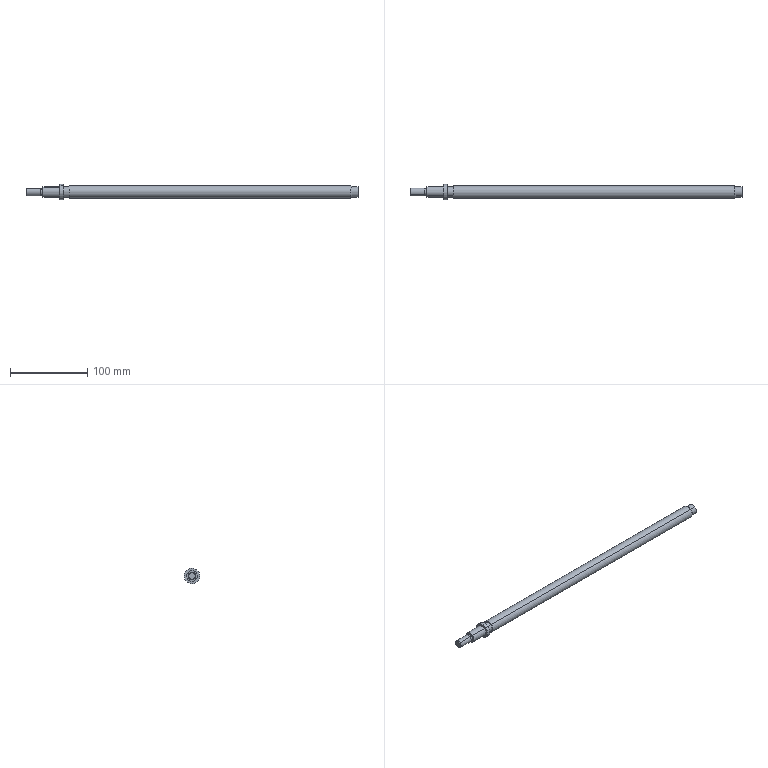Component | SolidWorks | 32FineAdjustmentLeadScrew-1 | 1 solid | 26 faces | box 430 x 20 x 20 mm | volume 81961 mm3 | cylinder 14 | plane 8 | cone 4 | commonest cylinder face diameters 13 x4 10 x2 8 x2 14 x2 20 x2 16 x2
STEP:
#1=COLOUR_RGB('',0.7922,0.8196,0.9333);
#2=FILL_AREA_STYLE_COLOUR('',#1);
#3=FILL_AREA_STYLE('',(#2));
#4=SURFACE_STYLE_FILL_AREA(#3);
#5=SURFACE_SIDE_STYLE('',(#4));
#6=SURFACE_STYLE_USAGE(.BOTH.,#5);
#7=PRESENTATION_STYLE_ASSIGNMENT((#6));
#8=CARTESIAN_POINT('',(7.008,2.405,-4.648));
#9=VERTEX_POINT('',#8);
#10=CARTESIAN_POINT('',(7.008,2.083,-4.25));
#11=VERTEX_POINT('',#10);
#12=CARTESIAN_POINT('',(7.008,2.244,-4.449));
#13=DIRECTION('',(-1.,-0.,0.));
#14=DIRECTION('',(0.,0.6286,-0.7777));
#15=AXIS2_PLACEMENT_3D('',#12,#13,#14);
#16=CIRCLE('',#15,0.2559);
#17=EDGE_CURVE('',#9,#11,#16,.T.);
#18=ORIENTED_EDGE('',*,*,#17,.F.);
#19=CARTESIAN_POINT('',(7.323,2.405,-4.648));
#20=VERTEX_POINT('',#19);
#21=CARTESIAN_POINT('',(7.008,2.405,-4.648));
#22=DIRECTION('',(1.,0.,-0.));
#23=VECTOR('',#22,39.37);
#24=LINE('',#21,#23);
#25=EDGE_CURVE('',#9,#20,#24,.T.);
#26=ORIENTED_EDGE('',*,*,#25,.T.);
#27=CARTESIAN_POINT('',(7.323,2.083,-4.25));
#28=VERTEX_POINT('',#27);
#29=CARTESIAN_POINT('',(7.323,2.244,-4.449));
#30=DIRECTION('',(-1.,-0.,0.));
#31=DIRECTION('',(0.,0.6286,-0.7777));
#32=AXIS2_PLACEMENT_3D('',#29,#30,#31);
#33=CIRCLE('',#32,0.2559);
#34=EDGE_CURVE('',#20,#28,#33,.T.);
#35=ORIENTED_EDGE('',*,*,#34,.T.);
#36=CARTESIAN_POINT('',(7.008,2.083,-4.25));
#37=DIRECTION('',(1.,0.,-0.));
#38=VECTOR('',#37,39.37);
#39=LINE('',#36,#38);
#40=EDGE_CURVE('',#11,#28,#39,.T.);
#41=ORIENTED_EDGE('',*,*,#40,.F.);
#42=EDGE_LOOP('',(#18,#26,#35,#41));
#43=FACE_OUTER_BOUND('',#42,.T.);
#44=CARTESIAN_POINT('',(7.008,2.244,-4.449));
#45=DIRECTION('',(1.,0.,-0.));
#46=DIRECTION('',(0.,-0.6286,0.7777));
#47=AXIS2_PLACEMENT_3D('',#44,#45,#46);
#48=CYLINDRICAL_SURFACE('',#47,0.2559);
#49=ADVANCED_FACE('',(#43),#48,.T.);
#50=CARTESIAN_POINT('',(7.008,2.415,-4.661));
#51=VERTEX_POINT('',#50);
#52=CARTESIAN_POINT('',(7.008,2.073,-4.237));
#53=VERTEX_POINT('',#52);
#54=CARTESIAN_POINT('',(7.008,2.244,-4.449));
#55=DIRECTION('',(-1.,-0.,0.));
#56=DIRECTION('',(0.,0.6286,-0.7777));
#57=AXIS2_PLACEMENT_3D('',#54,#55,#56);
#58=CIRCLE('',#57,0.2723);
#59=EDGE_CURVE('',#51,#53,#58,.T.);
#60=ORIENTED_EDGE('',*,*,#59,.T.);
#61=CARTESIAN_POINT('',(6.965,2.046,-4.204));
#62=VERTEX_POINT('',#61);
#63=CARTESIAN_POINT('',(7.008,2.073,-4.237));
#64=DIRECTION('',(-0.7071,-0.4445,0.5499));
#65=VECTOR('',#64,39.37);
#66=LINE('',#63,#65);
#67=EDGE_CURVE('',#53,#62,#66,.T.);
#68=ORIENTED_EDGE('',*,*,#67,.T.);
#69=CARTESIAN_POINT('',(6.965,2.442,-4.694));
#70=VERTEX_POINT('',#69);
#71=CARTESIAN_POINT('',(6.965,2.244,-4.449));
#72=DIRECTION('',(-1.,-0.,0.));
#73=DIRECTION('',(0.,0.6286,-0.7777));
#74=AXIS2_PLACEMENT_3D('',#71,#72,#73);
#75=CIRCLE('',#74,0.315);
#76=EDGE_CURVE('',#70,#62,#75,.T.);
#77=ORIENTED_EDGE('',*,*,#76,.F.);
#78=CARTESIAN_POINT('',(7.008,2.415,-4.661));
#79=DIRECTION('',(-0.7071,0.4445,-0.5499));
#80=VECTOR('',#79,39.37);
#81=LINE('',#78,#80);
#82=EDGE_CURVE('',#51,#70,#81,.T.);
#83=ORIENTED_EDGE('',*,*,#82,.F.);
#84=EDGE_LOOP('',(#60,#68,#77,#83));
#85=FACE_OUTER_BOUND('',#84,.T.);
#86=CARTESIAN_POINT('',(7.008,2.244,-4.449));
#87=DIRECTION('',(-1.,-0.,0.));
#88=DIRECTION('',(0.,0.6286,-0.7777));
#89=AXIS2_PLACEMENT_3D('',#86,#87,#88);
#90=CONICAL_SURFACE('',#89,0.2723,0.7854);
#91=ADVANCED_FACE('',(#85),#90,.T.);
#92=CARTESIAN_POINT('',(-9.606,2.14,-4.321));
#93=VERTEX_POINT('',#92);
#94=CARTESIAN_POINT('',(-9.606,2.348,-4.577));
#95=VERTEX_POINT('',#94);
#96=CARTESIAN_POINT('',(-9.606,2.244,-4.449));
#97=DIRECTION('',(1.,0.,-0.));
#98=DIRECTION('',(0.,-0.6286,0.7777));
#99=AXIS2_PLACEMENT_3D('',#96,#97,#98);
#100=CIRCLE('',#99,0.1649);
#101=EDGE_CURVE('',#93,#95,#100,.T.);
#102=ORIENTED_EDGE('',*,*,#101,.T.);
#103=CARTESIAN_POINT('',(-9.574,2.368,-4.602));
#104=VERTEX_POINT('',#103);
#105=CARTESIAN_POINT('',(-9.606,2.348,-4.577));
#106=DIRECTION('',(0.7071,0.4445,-0.5499));
#107=VECTOR('',#106,39.37);
#108=LINE('',#105,#107);
#109=EDGE_CURVE('',#95,#104,#108,.T.);
#110=ORIENTED_EDGE('',*,*,#109,.T.);
#111=CARTESIAN_POINT('',(-9.574,2.12,-4.296));
#112=VERTEX_POINT('',#111);
#113=CARTESIAN_POINT('',(-9.574,2.244,-4.449));
#114=DIRECTION('',(1.,0.,-0.));
#115=DIRECTION('',(0.,-0.6286,0.7777));
#116=AXIS2_PLACEMENT_3D('',#113,#114,#115);
#117=CIRCLE('',#116,0.1969);
#118=EDGE_CURVE('',#112,#104,#117,.T.);
#119=ORIENTED_EDGE('',*,*,#118,.F.);
#120=CARTESIAN_POINT('',(-9.606,2.14,-4.321));
#121=DIRECTION('',(0.7071,-0.4445,0.5499));
#122=VECTOR('',#121,39.37);
#123=LINE('',#120,#122);
#124=EDGE_CURVE('',#93,#112,#123,.T.);
#125=ORIENTED_EDGE('',*,*,#124,.F.);
#126=EDGE_LOOP('',(#102,#110,#119,#125));
#127=FACE_OUTER_BOUND('',#126,.T.);
#128=CARTESIAN_POINT('',(-9.606,2.244,-4.449));
#129=DIRECTION('',(1.,0.,-0.));
#130=DIRECTION('',(0.,-0.6286,0.7777));
#131=AXIS2_PLACEMENT_3D('',#128,#129,#130);
#132=CONICAL_SURFACE('',#131,0.1649,0.7854);
#133=ADVANCED_FACE('',(#127),#132,.T.);
#134=ORIENTED_EDGE('',*,*,#118,.T.);
#135=CARTESIAN_POINT('',(-8.858,2.368,-4.602));
#136=VERTEX_POINT('',#135);
#137=CARTESIAN_POINT('',(-9.606,2.368,-4.602));
#138=DIRECTION('',(1.,0.,-0.));
#139=VECTOR('',#138,39.37);
#140=LINE('',#137,#139);
#141=EDGE_CURVE('',#104,#136,#140,.T.);
#142=ORIENTED_EDGE('',*,*,#141,.T.);
#143=CARTESIAN_POINT('',(-8.858,2.12,-4.296));
#144=VERTEX_POINT('',#143);
#145=CARTESIAN_POINT('',(-8.858,2.244,-4.449));
#146=DIRECTION('',(-1.,-0.,0.));
#147=DIRECTION('',(0.,0.6286,-0.7777));
#148=AXIS2_PLACEMENT_3D('',#145,#146,#147);
#149=CIRCLE('',#148,0.1969);
#150=EDGE_CURVE('',#136,#144,#149,.T.);
#151=ORIENTED_EDGE('',*,*,#150,.T.);
#152=CARTESIAN_POINT('',(-9.606,2.12,-4.296));
#153=DIRECTION('',(1.,0.,-0.));
#154=VECTOR('',#153,39.37);
#155=LINE('',#152,#154);
#156=EDGE_CURVE('',#112,#144,#155,.T.);
#157=ORIENTED_EDGE('',*,*,#156,.F.);
#158=EDGE_LOOP('',(#134,#142,#151,#157));
#159=FACE_OUTER_BOUND('',#158,.T.);
#160=CARTESIAN_POINT('',(-9.606,2.244,-4.449));
#161=DIRECTION('',(1.,0.,-0.));
#162=DIRECTION('',(0.,-0.6286,0.7777));
#163=AXIS2_PLACEMENT_3D('',#160,#161,#162);
#164=CYLINDRICAL_SURFACE('',#163,0.1969);
#165=ADVANCED_FACE('',(#159),#164,.T.);
#166=CARTESIAN_POINT('',(-8.858,2.343,-4.571));
#167=VERTEX_POINT('',#166);
#168=CARTESIAN_POINT('',(-8.858,2.145,-4.326));
#169=VERTEX_POINT('',#168);
#170=CARTESIAN_POINT('',(-8.858,2.244,-4.449));
#171=DIRECTION('',(-1.,-0.,0.));
#172=DIRECTION('',(0.,0.6286,-0.7777));
#173=AXIS2_PLACEMENT_3D('',#170,#171,#172);
#174=CIRCLE('',#173,0.1575);
#175=EDGE_CURVE('',#167,#169,#174,.T.);
#176=ORIENTED_EDGE('',*,*,#175,.F.);
#177=CARTESIAN_POINT('',(-8.74,2.343,-4.571));
#178=VERTEX_POINT('',#177);
#179=CARTESIAN_POINT('',(-8.858,2.343,-4.571));
#180=DIRECTION('',(1.,0.,-0.));
#181=VECTOR('',#180,39.37);
#182=LINE('',#179,#181);
#183=EDGE_CURVE('',#167,#178,#182,.T.);
#184=ORIENTED_EDGE('',*,*,#183,.T.);
#185=CARTESIAN_POINT('',(-8.74,2.145,-4.326));
#186=VERTEX_POINT('',#185);
#187=CARTESIAN_POINT('',(-8.74,2.244,-4.449));
#188=DIRECTION('',(-1.,-0.,0.));
#189=DIRECTION('',(0.,0.6286,-0.7777));
#190=AXIS2_PLACEMENT_3D('',#187,#188,#189);
#191=CIRCLE('',#190,0.1575);
#192=EDGE_CURVE('',#178,#186,#191,.T.);
#193=ORIENTED_EDGE('',*,*,#192,.T.);
#194=CARTESIAN_POINT('',(-8.858,2.145,-4.326));
#195=DIRECTION('',(1.,0.,-0.));
#196=VECTOR('',#195,39.37);
#197=LINE('',#194,#196);
#198=EDGE_CURVE('',#169,#186,#197,.T.);
#199=ORIENTED_EDGE('',*,*,#198,.F.);
#200=EDGE_LOOP('',(#176,#184,#193,#199));
#201=FACE_OUTER_BOUND('',#200,.T.);
#202=CARTESIAN_POINT('',(-8.858,2.244,-4.449));
#203=DIRECTION('',(1.,0.,-0.));
#204=DIRECTION('',(0.,-0.6286,0.7777));
#205=AXIS2_PLACEMENT_3D('',#202,#203,#204);
#206=CYLINDRICAL_SURFACE('',#205,0.1575);
#207=ADVANCED_FACE('',(#201),#206,.T.);
#208=CARTESIAN_POINT('',(-8.74,2.417,-4.663));
#209=VERTEX_POINT('',#208);
#210=CARTESIAN_POINT('',(-8.74,2.071,-4.234));
#211=VERTEX_POINT('',#210);
#212=CARTESIAN_POINT('',(-8.74,2.244,-4.449));
#213=DIRECTION('',(-1.,-0.,0.));
#214=DIRECTION('',(0.,0.6286,-0.7777));
#215=AXIS2_PLACEMENT_3D('',#212,#213,#214);
#216=CIRCLE('',#215,0.2756);
#217=EDGE_CURVE('',#209,#211,#216,.T.);
#218=ORIENTED_EDGE('',*,*,#217,.F.);
#219=CARTESIAN_POINT('',(-7.874,2.417,-4.663));
#220=VERTEX_POINT('',#219);
#221=CARTESIAN_POINT('',(-8.74,2.417,-4.663));
#222=DIRECTION('',(1.,0.,-0.));
#223=VECTOR('',#222,39.37);
#224=LINE('',#221,#223);
#225=EDGE_CURVE('',#209,#220,#224,.T.);
#226=ORIENTED_EDGE('',*,*,#225,.T.);
#227=CARTESIAN_POINT('',(-7.874,2.071,-4.234));
#228=VERTEX_POINT('',#227);
#229=CARTESIAN_POINT('',(-7.874,2.244,-4.449));
#230=DIRECTION('',(-1.,-0.,0.));
#231=DIRECTION('',(0.,0.6286,-0.7777));
#232=AXIS2_PLACEMENT_3D('',#229,#230,#231);
#233=CIRCLE('',#232,0.2756);
#234=EDGE_CURVE('',#220,#228,#233,.T.);
#235=ORIENTED_EDGE('',*,*,#234,.T.);
#236=CARTESIAN_POINT('',(-8.74,2.071,-4.234));
#237=DIRECTION('',(1.,0.,-0.));
#238=VECTOR('',#237,39.37);
#239=LINE('',#236,#238);
#240=EDGE_CURVE('',#211,#228,#239,.T.);
#241=ORIENTED_EDGE('',*,*,#240,.F.);
#242=EDGE_LOOP('',(#218,#226,#235,#241));
#243=FACE_OUTER_BOUND('',#242,.T.);
#244=CARTESIAN_POINT('',(-8.74,2.244,-4.449));
#245=DIRECTION('',(1.,0.,-0.));
#246=DIRECTION('',(0.,-0.6286,0.7777));
#247=AXIS2_PLACEMENT_3D('',#244,#245,#246);
#248=CYLINDRICAL_SURFACE('',#247,0.2756);
#249=ADVANCED_FACE('',(#243),#248,.T.);
#250=CARTESIAN_POINT('',(-7.874,2.492,-4.755));
#251=VERTEX_POINT('',#250);
#252=CARTESIAN_POINT('',(-7.874,1.997,-4.143));
#253=VERTEX_POINT('',#252);
#254=CARTESIAN_POINT('',(-7.874,2.244,-4.449));
#255=DIRECTION('',(-1.,-0.,0.));
#256=DIRECTION('',(0.,0.6286,-0.7777));
#257=AXIS2_PLACEMENT_3D('',#254,#255,#256);
#258=CIRCLE('',#257,0.3937);
#259=EDGE_CURVE('',#251,#253,#258,.T.);
#260=ORIENTED_EDGE('',*,*,#259,.F.);
#261=CARTESIAN_POINT('',(-7.717,2.492,-4.755));
#262=VERTEX_POINT('',#261);
#263=CARTESIAN_POINT('',(-7.874,2.492,-4.755));
#264=DIRECTION('',(1.,0.,-0.));
#265=VECTOR('',#264,39.37);
#266=LINE('',#263,#265);
#267=EDGE_CURVE('',#251,#262,#266,.T.);
#268=ORIENTED_EDGE('',*,*,#267,.T.);
#269=CARTESIAN_POINT('',(-7.717,1.997,-4.143));
#270=VERTEX_POINT('',#269);
#271=CARTESIAN_POINT('',(-7.717,2.244,-4.449));
#272=DIRECTION('',(-1.,-0.,0.));
#273=DIRECTION('',(0.,0.6286,-0.7777));
#274=AXIS2_PLACEMENT_3D('',#271,#272,#273);
#275=CIRCLE('',#274,0.3937);
#276=EDGE_CURVE('',#262,#270,#275,.T.);
#277=ORIENTED_EDGE('',*,*,#276,.T.);
#278=CARTESIAN_POINT('',(-7.874,1.997,-4.143));
#279=DIRECTION('',(1.,0.,-0.));
#280=VECTOR('',#279,39.37);
#281=LINE('',#278,#280);
#282=EDGE_CURVE('',#253,#270,#281,.T.);
#283=ORIENTED_EDGE('',*,*,#282,.F.);
#284=EDGE_LOOP('',(#260,#268,#277,#283));
#285=FACE_OUTER_BOUND('',#284,.T.);
#286=CARTESIAN_POINT('',(-7.874,2.244,-4.449));
#287=DIRECTION('',(1.,0.,-0.));
#288=DIRECTION('',(0.,-0.6286,0.7777));
#289=AXIS2_PLACEMENT_3D('',#286,#287,#288);
#290=CYLINDRICAL_SURFACE('',#289,0.3937);
#291=ADVANCED_FACE('',(#285),#290,.T.);
#292=CARTESIAN_POINT('',(-7.717,2.405,-4.648));
#293=VERTEX_POINT('',#292);
#294=CARTESIAN_POINT('',(-7.717,2.083,-4.25));
#295=VERTEX_POINT('',#294);
#296=CARTESIAN_POINT('',(-7.717,2.244,-4.449));
#297=DIRECTION('',(-1.,-0.,0.));
#298=DIRECTION('',(0.,0.6286,-0.7777));
#299=AXIS2_PLACEMENT_3D('',#296,#297,#298);
#300=CIRCLE('',#299,0.2559);
#301=EDGE_CURVE('',#293,#295,#300,.T.);
#302=ORIENTED_EDGE('',*,*,#301,.F.);
#303=CARTESIAN_POINT('',(-7.402,2.405,-4.648));
#304=VERTEX_POINT('',#303);
#305=CARTESIAN_POINT('',(-7.717,2.405,-4.648));
#306=DIRECTION('',(1.,0.,-0.));
#307=VECTOR('',#306,39.37);
#308=LINE('',#305,#307);
#309=EDGE_CURVE('',#293,#304,#308,.T.);
#310=ORIENTED_EDGE('',*,*,#309,.T.);
#311=CARTESIAN_POINT('',(-7.402,2.083,-4.25));
#312=VERTEX_POINT('',#311);
#313=CARTESIAN_POINT('',(-7.402,2.244,-4.449));
#314=DIRECTION('',(-1.,-0.,0.));
#315=DIRECTION('',(0.,0.6286,-0.7777));
#316=AXIS2_PLACEMENT_3D('',#313,#314,#315);
#317=CIRCLE('',#316,0.2559);
#318=EDGE_CURVE('',#304,#312,#317,.T.);
#319=ORIENTED_EDGE('',*,*,#318,.T.);
#320=CARTESIAN_POINT('',(-7.717,2.083,-4.25));
#321=DIRECTION('',(1.,0.,-0.));
#322=VECTOR('',#321,39.37);
#323=LINE('',#320,#322);
#324=EDGE_CURVE('',#295,#312,#323,.T.);
#325=ORIENTED_EDGE('',*,*,#324,.F.);
#326=EDGE_LOOP('',(#302,#310,#319,#325));
#327=FACE_OUTER_BOUND('',#326,.T.);
#328=CARTESIAN_POINT('',(-7.717,2.244,-4.449));
#329=DIRECTION('',(1.,0.,-0.));
#330=DIRECTION('',(0.,-0.6286,0.7777));
#331=AXIS2_PLACEMENT_3D('',#328,#329,#330);
#332=CYLINDRICAL_SURFACE('',#331,0.2559);
#333=ADVANCED_FACE('',(#327),#332,.T.);
#334=CARTESIAN_POINT('',(-7.402,2.442,-4.694));
#335=VERTEX_POINT('',#334);
#336=CARTESIAN_POINT('',(-7.402,2.046,-4.204));
#337=VERTEX_POINT('',#336);
#338=CARTESIAN_POINT('',(-7.402,2.244,-4.449));
#339=DIRECTION('',(-1.,-0.,0.));
#340=DIRECTION('',(0.,0.6286,-0.7777));
#341=AXIS2_PLACEMENT_3D('',#338,#339,#340);
#342=CIRCLE('',#341,0.315);
#343=EDGE_CURVE('',#335,#337,#342,.T.);
#344=ORIENTED_EDGE('',*,*,#343,.F.);
#345=CARTESIAN_POINT('',(-7.402,2.442,-4.694));
#346=DIRECTION('',(1.,0.,-0.));
#347=VECTOR('',#346,39.37);
#348=LINE('',#345,#347);
#349=EDGE_CURVE('',#335,#70,#348,.T.);
#350=ORIENTED_EDGE('',*,*,#349,.T.);
#351=ORIENTED_EDGE('',*,*,#76,.T.);
#352=CARTESIAN_POINT('',(-7.402,2.046,-4.204));
#353=DIRECTION('',(1.,0.,-0.));
#354=VECTOR('',#353,39.37);
#355=LINE('',#352,#354);
#356=EDGE_CURVE('',#337,#62,#355,.T.);
#357=ORIENTED_EDGE('',*,*,#356,.F.);
#358=EDGE_LOOP('',(#344,#350,#351,#357));
#359=FACE_OUTER_BOUND('',#358,.T.);
#360=CARTESIAN_POINT('',(-7.402,2.244,-4.449));
#361=DIRECTION('',(1.,0.,-0.));
#362=DIRECTION('',(0.,-0.6286,0.7777));
#363=AXIS2_PLACEMENT_3D('',#360,#361,#362);
#364=CYLINDRICAL_SURFACE('',#363,0.315);
#365=ADVANCED_FACE('',(#359),#364,.T.);
#366=ORIENTED_EDGE('',*,*,#349,.F.);
#367=CARTESIAN_POINT('',(-7.402,2.244,-4.449));
#368=DIRECTION('',(-1.,-0.,0.));
#369=DIRECTION('',(0.,0.6286,-0.7777));
#370=AXIS2_PLACEMENT_3D('',#367,#368,#369);
#371=CIRCLE('',#370,0.315);
#372=EDGE_CURVE('',#337,#335,#371,.T.);
#373=ORIENTED_EDGE('',*,*,#372,.F.);
#374=ORIENTED_EDGE('',*,*,#356,.T.);
#375=CARTESIAN_POINT('',(6.965,2.244,-4.449));
#376=DIRECTION('',(-1.,-0.,0.));
#377=DIRECTION('',(0.,0.6286,-0.7777));
#378=AXIS2_PLACEMENT_3D('',#375,#376,#377);
#379=CIRCLE('',#378,0.315);
#380=EDGE_CURVE('',#62,#70,#379,.T.);
#381=ORIENTED_EDGE('',*,*,#380,.T.);
#382=EDGE_LOOP('',(#366,#373,#374,#381));
#383=FACE_OUTER_BOUND('',#382,.T.);
#384=CARTESIAN_POINT('',(-7.402,2.244,-4.449));
#385=DIRECTION('',(1.,0.,-0.));
#386=DIRECTION('',(0.,-0.6286,0.7777));
#387=AXIS2_PLACEMENT_3D('',#384,#385,#386);
#388=CYLINDRICAL_SURFACE('',#387,0.315);
#389=ADVANCED_FACE('',(#383),#388,.T.);
#390=CARTESIAN_POINT('',(-7.402,2.244,-4.449));
#391=DIRECTION('',(-1.,-0.,0.));
#392=DIRECTION('',(0.,0.6286,-0.7777));
#393=AXIS2_PLACEMENT_3D('',#390,#391,#392);
#394=CIRCLE('',#393,0.2559);
#395=EDGE_CURVE('',#312,#304,#394,.T.);
#396=ORIENTED_EDGE('',*,*,#395,.F.);
#397=ORIENTED_EDGE('',*,*,#318,.F.);
#398=EDGE_LOOP('',(#396,#397));
#399=FACE_BOUND('',#398,.T.);
#400=ORIENTED_EDGE('',*,*,#372,.T.);
#401=ORIENTED_EDGE('',*,*,#343,.T.);
#402=EDGE_LOOP('',(#400,#401));
#403=FACE_OUTER_BOUND('',#402,.T.);
#404=CARTESIAN_POINT('',(-7.402,2.244,-4.449));
#405=DIRECTION('',(-1.,-0.,0.));
#406=DIRECTION('',(-0.,0.6286,-0.7777));
#407=AXIS2_PLACEMENT_3D('',#404,#405,#406);
#408=PLANE('',#407);
#409=ADVANCED_FACE('',(#399,#403),#408,.T.);
#410=ORIENTED_EDGE('',*,*,#309,.F.);
#411=CARTESIAN_POINT('',(-7.717,2.244,-4.449));
#412=DIRECTION('',(-1.,-0.,0.));
#413=DIRECTION('',(0.,0.6286,-0.7777));
#414=AXIS2_PLACEMENT_3D('',#411,#412,#413);
#415=CIRCLE('',#414,0.2559);
#416=EDGE_CURVE('',#295,#293,#415,.T.);
#417=ORIENTED_EDGE('',*,*,#416,.F.);
#418=ORIENTED_EDGE('',*,*,#324,.T.);
#419=ORIENTED_EDGE('',*,*,#395,.T.);
#420=EDGE_LOOP('',(#410,#417,#418,#419));
#421=FACE_OUTER_BOUND('',#420,.T.);
#422=CARTESIAN_POINT('',(-7.717,2.244,-4.449));
#423=DIRECTION('',(1.,0.,-0.));
#424=DIRECTION('',(0.,-0.6286,0.7777));
#425=AXIS2_PLACEMENT_3D('',#422,#423,#424);
#426=CYLINDRICAL_SURFACE('',#425,0.2559);
#427=ADVANCED_FACE('',(#421),#426,.T.);
#428=ORIENTED_EDGE('',*,*,#267,.F.);
#429=CARTESIAN_POINT('',(-7.874,2.244,-4.449));
#430=DIRECTION('',(-1.,-0.,0.));
#431=DIRECTION('',(0.,0.6286,-0.7777));
#432=AXIS2_PLACEMENT_3D('',#429,#430,#431);
#433=CIRCLE('',#432,0.3937);
#434=EDGE_CURVE('',#253,#251,#433,.T.);
#435=ORIENTED_EDGE('',*,*,#434,.F.);
#436=ORIENTED_EDGE('',*,*,#282,.T.);
#437=CARTESIAN_POINT('',(-7.717,2.244,-4.449));
#438=DIRECTION('',(-1.,-0.,0.));
#439=DIRECTION('',(0.,0.6286,-0.7777));
#440=AXIS2_PLACEMENT_3D('',#437,#438,#439);
#441=CIRCLE('',#440,0.3937);
#442=EDGE_CURVE('',#270,#262,#441,.T.);
#443=ORIENTED_EDGE('',*,*,#442,.T.);
#444=EDGE_LOOP('',(#428,#435,#436,#443));
#445=FACE_OUTER_BOUND('',#444,.T.);
#446=CARTESIAN_POINT('',(-7.874,2.244,-4.449));
#447=DIRECTION('',(1.,0.,-0.));
#448=DIRECTION('',(0.,-0.6286,0.7777));
#449=AXIS2_PLACEMENT_3D('',#446,#447,#448);
#450=CYLINDRICAL_SURFACE('',#449,0.3937);
#451=ADVANCED_FACE('',(#445),#450,.T.);
#452=CARTESIAN_POINT('',(-7.874,2.244,-4.449));
#453=DIRECTION('',(-1.,-0.,0.));
#454=DIRECTION('',(0.,0.6286,-0.7777));
#455=AXIS2_PLACEMENT_3D('',#452,#453,#454);
#456=CIRCLE('',#455,0.2756);
#457=EDGE_CURVE('',#228,#220,#456,.T.);
#458=ORIENTED_EDGE('',*,*,#457,.F.);
#459=ORIENTED_EDGE('',*,*,#234,.F.);
#460=EDGE_LOOP('',(#458,#459));
#461=FACE_BOUND('',#460,.T.);
#462=ORIENTED_EDGE('',*,*,#434,.T.);
#463=ORIENTED_EDGE('',*,*,#259,.T.);
#464=EDGE_LOOP('',(#462,#463));
#465=FACE_OUTER_BOUND('',#464,.T.);
#466=CARTESIAN_POINT('',(-7.874,2.244,-4.449));
#467=DIRECTION('',(-1.,-0.,0.));
#468=DIRECTION('',(-0.,0.6286,-0.7777));
#469=AXIS2_PLACEMENT_3D('',#466,#467,#468);
#470=PLANE('',#469);
#471=ADVANCED_FACE('',(#461,#465),#470,.T.);
#472=ORIENTED_EDGE('',*,*,#416,.T.);
#473=ORIENTED_EDGE('',*,*,#301,.T.);
#474=EDGE_LOOP('',(#472,#473));
#475=FACE_BOUND('',#474,.T.);
#476=ORIENTED_EDGE('',*,*,#442,.F.);
#477=ORIENTED_EDGE('',*,*,#276,.F.);
#478=EDGE_LOOP('',(#476,#477));
#479=FACE_OUTER_BOUND('',#478,.T.);
#480=CARTESIAN_POINT('',(-7.717,2.244,-4.449));
#481=DIRECTION('',(-1.,-0.,0.));
#482=DIRECTION('',(-0.,0.6286,-0.7777));
#483=AXIS2_PLACEMENT_3D('',#480,#481,#482);
#484=PLANE('',#483);
#485=ADVANCED_FACE('',(#475,#479),#484,.F.);
#486=ORIENTED_EDGE('',*,*,#225,.F.);
#487=CARTESIAN_POINT('',(-8.74,2.244,-4.449));
#488=DIRECTION('',(-1.,-0.,0.));
#489=DIRECTION('',(0.,0.6286,-0.7777));
#490=AXIS2_PLACEMENT_3D('',#487,#488,#489);
#491=CIRCLE('',#490,0.2756);
#492=EDGE_CURVE('',#211,#209,#491,.T.);
#493=ORIENTED_EDGE('',*,*,#492,.F.);
#494=ORIENTED_EDGE('',*,*,#240,.T.);
#495=ORIENTED_EDGE('',*,*,#457,.T.);
#496=EDGE_LOOP('',(#486,#493,#494,#495));
#497=FACE_OUTER_BOUND('',#496,.T.);
#498=CARTESIAN_POINT('',(-8.74,2.244,-4.449));
#499=DIRECTION('',(1.,0.,-0.));
#500=DIRECTION('',(0.,-0.6286,0.7777));
#501=AXIS2_PLACEMENT_3D('',#498,#499,#500);
#502=CYLINDRICAL_SURFACE('',#501,0.2756);
#503=ADVANCED_FACE('',(#497),#502,.T.);
#504=CARTESIAN_POINT('',(-8.74,2.244,-4.449));
#505=DIRECTION('',(-1.,-0.,0.));
#506=DIRECTION('',(0.,0.6286,-0.7777));
#507=AXIS2_PLACEMENT_3D('',#504,#505,#506);
#508=CIRCLE('',#507,0.1575);
#509=EDGE_CURVE('',#186,#178,#508,.T.);
#510=ORIENTED_EDGE('',*,*,#509,.F.);
#511=ORIENTED_EDGE('',*,*,#192,.F.);
#512=EDGE_LOOP('',(#510,#511));
#513=FACE_BOUND('',#512,.T.);
#514=ORIENTED_EDGE('',*,*,#492,.T.);
#515=ORIENTED_EDGE('',*,*,#217,.T.);
#516=EDGE_LOOP('',(#514,#515));
#517=FACE_OUTER_BOUND('',#516,.T.);
#518=CARTESIAN_POINT('',(-8.74,2.244,-4.449));
#519=DIRECTION('',(-1.,-0.,0.));
#520=DIRECTION('',(-0.,0.6286,-0.7777));
#521=AXIS2_PLACEMENT_3D('',#518,#519,#520);
#522=PLANE('',#521);
#523=ADVANCED_FACE('',(#513,#517),#522,.T.);
#524=ORIENTED_EDGE('',*,*,#183,.F.);
#525=CARTESIAN_POINT('',(-8.858,2.244,-4.449));
#526=DIRECTION('',(-1.,-0.,0.));
#527=DIRECTION('',(0.,0.6286,-0.7777));
#528=AXIS2_PLACEMENT_3D('',#525,#526,#527);
#529=CIRCLE('',#528,0.1575);
#530=EDGE_CURVE('',#169,#167,#529,.T.);
#531=ORIENTED_EDGE('',*,*,#530,.F.);
#532=ORIENTED_EDGE('',*,*,#198,.T.);
#533=ORIENTED_EDGE('',*,*,#509,.T.);
#534=EDGE_LOOP('',(#524,#531,#532,#533));
#535=FACE_OUTER_BOUND('',#534,.T.);
#536=CARTESIAN_POINT('',(-8.858,2.244,-4.449));
#537=DIRECTION('',(1.,0.,-0.));
#538=DIRECTION('',(0.,-0.6286,0.7777));
#539=AXIS2_PLACEMENT_3D('',#536,#537,#538);
#540=CYLINDRICAL_SURFACE('',#539,0.1575);
#541=ADVANCED_FACE('',(#535),#540,.T.);
#542=ORIENTED_EDGE('',*,*,#141,.F.);
#543=CARTESIAN_POINT('',(-9.574,2.244,-4.449));
#544=DIRECTION('',(1.,0.,-0.));
#545=DIRECTION('',(0.,-0.6286,0.7777));
#546=AXIS2_PLACEMENT_3D('',#543,#544,#545);
#547=CIRCLE('',#546,0.1969);
#548=EDGE_CURVE('',#104,#112,#547,.T.);
#549=ORIENTED_EDGE('',*,*,#548,.T.);
#550=ORIENTED_EDGE('',*,*,#156,.T.);
#551=CARTESIAN_POINT('',(-8.858,2.244,-4.449));
#552=DIRECTION('',(-1.,-0.,0.));
#553=DIRECTION('',(0.,0.6286,-0.7777));
#554=AXIS2_PLACEMENT_3D('',#551,#552,#553);
#555=CIRCLE('',#554,0.1969);
#556=EDGE_CURVE('',#144,#136,#555,.T.);
#557=ORIENTED_EDGE('',*,*,#556,.T.);
#558=EDGE_LOOP('',(#542,#549,#550,#557));
#559=FACE_OUTER_BOUND('',#558,.T.);
#560=CARTESIAN_POINT('',(-9.606,2.244,-4.449));
#561=DIRECTION('',(1.,0.,-0.));
#562=DIRECTION('',(0.,-0.6286,0.7777));
#563=AXIS2_PLACEMENT_3D('',#560,#561,#562);
#564=CYLINDRICAL_SURFACE('',#563,0.1969);
#565=ADVANCED_FACE('',(#559),#564,.T.);
#566=ORIENTED_EDGE('',*,*,#530,.T.);
#567=ORIENTED_EDGE('',*,*,#175,.T.);
#568=EDGE_LOOP('',(#566,#567));
#569=FACE_BOUND('',#568,.T.);
#570=ORIENTED_EDGE('',*,*,#556,.F.);
#571=ORIENTED_EDGE('',*,*,#150,.F.);
#572=EDGE_LOOP('',(#570,#571));
#573=FACE_OUTER_BOUND('',#572,.T.);
#574=CARTESIAN_POINT('',(-8.858,2.244,-4.449));
#575=DIRECTION('',(-1.,-0.,0.));
#576=DIRECTION('',(-0.,0.6286,-0.7777));
#577=AXIS2_PLACEMENT_3D('',#574,#575,#576);
#578=PLANE('',#577);
#579=ADVANCED_FACE('',(#569,#573),#578,.F.);
#580=ORIENTED_EDGE('',*,*,#109,.F.);
#581=CARTESIAN_POINT('',(-9.606,2.244,-4.449));
#582=DIRECTION('',(1.,0.,-0.));
#583=DIRECTION('',(0.,-0.6286,0.7777));
#584=AXIS2_PLACEMENT_3D('',#581,#582,#583);
#585=CIRCLE('',#584,0.1649);
#586=EDGE_CURVE('',#95,#93,#585,.T.);
#587=ORIENTED_EDGE('',*,*,#586,.T.);
#588=ORIENTED_EDGE('',*,*,#124,.T.);
#589=ORIENTED_EDGE('',*,*,#548,.F.);
#590=EDGE_LOOP('',(#580,#587,#588,#589));
#591=FACE_OUTER_BOUND('',#590,.T.);
#592=CARTESIAN_POINT('',(-9.606,2.244,-4.449));
#593=DIRECTION('',(1.,0.,-0.));
#594=DIRECTION('',(0.,-0.6286,0.7777));
#595=AXIS2_PLACEMENT_3D('',#592,#593,#594);
#596=CONICAL_SURFACE('',#595,0.1649,0.7854);
#597=ADVANCED_FACE('',(#591),#596,.T.);
#598=ORIENTED_EDGE('',*,*,#101,.F.);
#599=ORIENTED_EDGE('',*,*,#586,.F.);
#600=EDGE_LOOP('',(#598,#599));
#601=FACE_OUTER_BOUND('',#600,.T.);
#602=CARTESIAN_POINT('',(-9.606,2.244,-4.449));
#603=DIRECTION('',(-1.,-0.,0.));
#604=DIRECTION('',(-0.,0.6286,-0.7777));
#605=AXIS2_PLACEMENT_3D('',#602,#603,#604);
#606=PLANE('',#605);
#607=ADVANCED_FACE('',(#601),#606,.T.);
#608=ORIENTED_EDGE('',*,*,#67,.F.);
#609=CARTESIAN_POINT('',(7.008,2.244,-4.449));
#610=DIRECTION('',(-1.,-0.,0.));
#611=DIRECTION('',(0.,0.6286,-0.7777));
#612=AXIS2_PLACEMENT_3D('',#609,#610,#611);
#613=CIRCLE('',#612,0.2723);
#614=EDGE_CURVE('',#53,#51,#613,.T.);
#615=ORIENTED_EDGE('',*,*,#614,.T.);
#616=ORIENTED_EDGE('',*,*,#82,.T.);
#617=ORIENTED_EDGE('',*,*,#380,.F.);
#618=EDGE_LOOP('',(#608,#615,#616,#617));
#619=FACE_OUTER_BOUND('',#618,.T.);
#620=CARTESIAN_POINT('',(7.008,2.244,-4.449));
#621=DIRECTION('',(-1.,-0.,0.));
#622=DIRECTION('',(0.,0.6286,-0.7777));
#623=AXIS2_PLACEMENT_3D('',#620,#621,#622);
#624=CONICAL_SURFACE('',#623,0.2723,0.7854);
#625=ADVANCED_FACE('',(#619),#624,.T.);
#626=CARTESIAN_POINT('',(7.323,2.244,-4.449));
#627=DIRECTION('',(-1.,-0.,0.));
#628=DIRECTION('',(0.,0.6286,-0.7777));
#629=AXIS2_PLACEMENT_3D('',#626,#627,#628);
#630=CIRCLE('',#629,0.2559);
#631=EDGE_CURVE('',#28,#20,#630,.T.);
#632=ORIENTED_EDGE('',*,*,#631,.F.);
#633=ORIENTED_EDGE('',*,*,#34,.F.);
#634=EDGE_LOOP('',(#632,#633));
#635=FACE_OUTER_BOUND('',#634,.T.);
#636=CARTESIAN_POINT('',(7.323,2.244,-4.449));
#637=DIRECTION('',(-1.,-0.,0.));
#638=DIRECTION('',(-0.,0.6286,-0.7777));
#639=AXIS2_PLACEMENT_3D('',#636,#637,#638);
#640=PLANE('',#639);
#641=ADVANCED_FACE('',(#635),#640,.F.);
#642=ORIENTED_EDGE('',*,*,#25,.F.);
#643=CARTESIAN_POINT('',(7.008,2.244,-4.449));
#644=DIRECTION('',(-1.,-0.,0.));
#645=DIRECTION('',(0.,0.6286,-0.7777));
#646=AXIS2_PLACEMENT_3D('',#643,#644,#645);
#647=CIRCLE('',#646,0.2559);
#648=EDGE_CURVE('',#11,#9,#647,.T.);
#649=ORIENTED_EDGE('',*,*,#648,.F.);
#650=ORIENTED_EDGE('',*,*,#40,.T.);
#651=ORIENTED_EDGE('',*,*,#631,.T.);
#652=EDGE_LOOP('',(#642,#649,#650,#651));
#653=FACE_OUTER_BOUND('',#652,.T.);
#654=CARTESIAN_POINT('',(7.008,2.244,-4.449));
#655=DIRECTION('',(1.,0.,-0.));
#656=DIRECTION('',(0.,-0.6286,0.7777));
#657=AXIS2_PLACEMENT_3D('',#654,#655,#656);
#658=CYLINDRICAL_SURFACE('',#657,0.2559);
#659=ADVANCED_FACE('',(#653),#658,.T.);
#660=ORIENTED_EDGE('',*,*,#648,.T.);
#661=ORIENTED_EDGE('',*,*,#17,.T.);
#662=EDGE_LOOP('',(#660,#661));
#663=FACE_BOUND('',#662,.T.);
#664=ORIENTED_EDGE('',*,*,#59,.F.);
#665=ORIENTED_EDGE('',*,*,#614,.F.);
#666=EDGE_LOOP('',(#664,#665));
#667=FACE_OUTER_BOUND('',#666,.T.);
#668=CARTESIAN_POINT('',(7.008,2.244,-4.449));
#669=DIRECTION('',(-1.,-0.,0.));
#670=DIRECTION('',(-0.,0.6286,-0.7777));
#671=AXIS2_PLACEMENT_3D('',#668,#669,#670);
#672=PLANE('',#671);
#673=ADVANCED_FACE('',(#663,#667),#672,.F.);
#674=CLOSED_SHELL('',(#49,#91,#133,#165,#207,#249,#291,#333,#365,#389,#409,#427,#451,#471,#485,#503,#523,#541,#565,#579,#597,#607,#625,#641,#659,#673));
#675=MANIFOLD_SOLID_BREP('',#674);
#676=STYLED_ITEM('',(#7),#675);
#677=(LENGTH_UNIT()NAMED_UNIT(*)SI_UNIT($,.METRE.));
#678=LENGTH_MEASURE_WITH_UNIT(LENGTH_MEASURE(0.0254),#677);
#679=DIMENSIONAL_EXPONENTS(1.,0.,0.,0.,0.,0.,0.);
#680=(CONVERSION_BASED_UNIT('',#678)LENGTH_UNIT()NAMED_UNIT(#679));
#681=UNCERTAINTY_MEASURE_WITH_UNIT(LENGTH_MEASURE(0.00001),#680,'','');
#682=(NAMED_UNIT(*)PLANE_ANGLE_UNIT()SI_UNIT($,.RADIAN.));
#683=(NAMED_UNIT(*)SI_UNIT($,.STERADIAN.)SOLID_ANGLE_UNIT());
#684=(GEOMETRIC_REPRESENTATION_CONTEXT(3)GLOBAL_UNCERTAINTY_ASSIGNED_CONTEXT((#681))GLOBAL_UNIT_ASSIGNED_CONTEXT((#680,#682,#683))REPRESENTATION_CONTEXT('',''));
#685=MECHANICAL_DESIGN_GEOMETRIC_PRESENTATION_REPRESENTATION('',(#676),#684);
#686=PRESENTATION_LAYER_ASSIGNMENT('','',(#676));
#687=CARTESIAN_POINT('',(0.,0.,0.));
#688=DIRECTION('',(0.,0.,1.));
#689=DIRECTION('',(1.,0.,0.));
#690=AXIS2_PLACEMENT_3D('',#687,#688,#689);
#691=(LENGTH_UNIT()NAMED_UNIT(*)SI_UNIT($,.METRE.));
#692=LENGTH_MEASURE_WITH_UNIT(LENGTH_MEASURE(0.0254),#691);
#693=DIMENSIONAL_EXPONENTS(1.,0.,0.,0.,0.,0.,0.);
#694=(CONVERSION_BASED_UNIT('',#692)LENGTH_UNIT()NAMED_UNIT(#693));
#695=UNCERTAINTY_MEASURE_WITH_UNIT(LENGTH_MEASURE(0.00001),#694,'','');
#696=(NAMED_UNIT(*)PLANE_ANGLE_UNIT()SI_UNIT($,.RADIAN.));
#697=(NAMED_UNIT(*)SI_UNIT($,.STERADIAN.)SOLID_ANGLE_UNIT());
#698=(GEOMETRIC_REPRESENTATION_CONTEXT(3)GLOBAL_UNCERTAINTY_ASSIGNED_CONTEXT((#695))GLOBAL_UNIT_ASSIGNED_CONTEXT((#694,#696,#697))REPRESENTATION_CONTEXT('',''));
#699=ADVANCED_BREP_SHAPE_REPRESENTATION('',(#675,#690),#698);